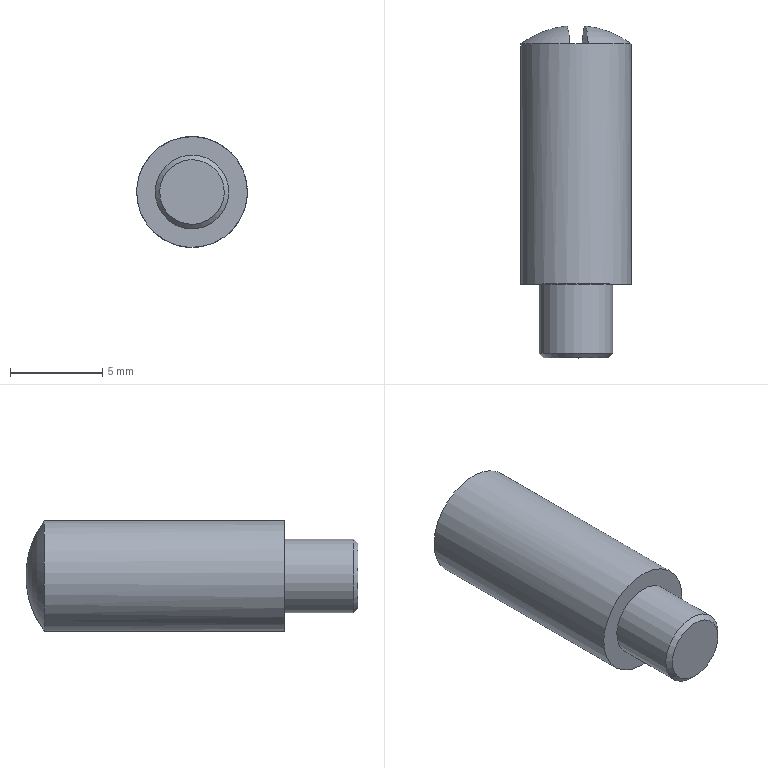Component | NX | CONN_PIN | 1 solid | 10 faces | box 6 x 17.97 x 6 mm | volume 428 mm3 | plane 5 | sphere 2 | cylinder 2 | cone 1 | commonest cylinder face diameters 4 x1 6 x1
STEP:
#1=CARTESIAN_POINT('',(0.,0.,0.));
#2=DIRECTION('',(0.,0.,1.));
#3=DIRECTION('',(1.,0.,0.));
#4=AXIS2_PLACEMENT_3D('',#1,#2,#3);
#5=CARTESIAN_POINT('',(-0.6646,-1.5,87.196));
#6=VERTEX_POINT('',#5);
#7=CARTESIAN_POINT('',(-0.3339,-1.5,93.103));
#8=VERTEX_POINT('',#7);
#9=CARTESIAN_POINT('',(-0.4992,-5.5,90.149));
#10=DIRECTION('',(0.9984,0.,-0.05589));
#11=DIRECTION('',(0.05589,0.,0.9984));
#12=AXIS2_PLACEMENT_3D('',#9,#10,#11);
#13=CIRCLE('',#12,4.975);
#14=CARTESIAN_POINT('',(-0.,-5.5,90.121));
#15=DIRECTION('',(-0.,1.,0.));
#16=DIRECTION('',(-0.05589,-0.,-0.9984));
#17=AXIS2_PLACEMENT_3D('',#14,#15,#16);
#18=SPHERICAL_SURFACE('',#17,5.);
#19=CARTESIAN_POINT('',(0.1674,0.9273));
#20=CARTESIAN_POINT('',(0.1718,0.9463));
#21=CARTESIAN_POINT('',(0.1811,0.9843));
#22=CARTESIAN_POINT('',(0.1985,1.041));
#23=CARTESIAN_POINT('',(0.2203,1.098));
#24=CARTESIAN_POINT('',(0.2482,1.154));
#25=CARTESIAN_POINT('',(0.2849,1.21));
#26=CARTESIAN_POINT('',(0.335,1.265));
#27=CARTESIAN_POINT('',(0.4066,1.319));
#28=CARTESIAN_POINT('',(0.5152,1.371));
#29=CARTESIAN_POINT('',(0.6936,1.419));
#30=CARTESIAN_POINT('',(1.007,1.459));
#31=CARTESIAN_POINT('',(1.571,1.477));
#32=CARTESIAN_POINT('',(2.135,1.459));
#33=CARTESIAN_POINT('',(2.448,1.419));
#34=CARTESIAN_POINT('',(2.626,1.371));
#35=CARTESIAN_POINT('',(2.735,1.319));
#36=CARTESIAN_POINT('',(2.807,1.265));
#37=CARTESIAN_POINT('',(2.857,1.21));
#38=CARTESIAN_POINT('',(2.893,1.154));
#39=CARTESIAN_POINT('',(2.921,1.098));
#40=CARTESIAN_POINT('',(2.943,1.041));
#41=CARTESIAN_POINT('',(2.96,0.9843));
#42=CARTESIAN_POINT('',(2.97,0.9463));
#43=CARTESIAN_POINT('',(2.974,0.9273));
#44=B_SPLINE_CURVE_WITH_KNOTS('',3,(#19,#20,#21,#22,#23,#24,#25,#26,#27,#28,#29,#30,#31,#32,#33,#34,#35,#36,#37,#38,#39,#40,#41,#42,#43),.UNSPECIFIED.,.F.,.F.,(4,1,1,1,1,1,1,1,1,1,1,1,1,1,1,1,1,1,1,1,1,1,4),(4.076,4.134,4.191,4.249,4.307,4.365,4.423,4.481,4.539,4.597,4.655,4.712,4.77,4.828,4.886,4.944,5.002,5.06,5.118,5.175,5.233,5.291,5.349),.QUASI_UNIFORM_KNOTS.);
#45=(GEOMETRIC_REPRESENTATION_CONTEXT(2)PARAMETRIC_REPRESENTATION_CONTEXT()REPRESENTATION_CONTEXT('',''));
#46=DEFINITIONAL_REPRESENTATION('',(#44),#45);
#47=PCURVE('',#18,#46);
#48=CARTESIAN_POINT('',(-0.1791,-0.5,95.868));
#49=DIRECTION('',(-0.9984,0.,0.05589));
#50=DIRECTION('',(0.05589,0.,0.9984));
#51=AXIS2_PLACEMENT_3D('',#48,#49,#50);
#52=PLANE('',#51);
#53=CARTESIAN_POINT('',(-0.7532,-5.));
#54=CARTESIAN_POINT('',(-0.7532,-13.617));
#55=CARTESIAN_POINT('',(-8.216,-9.308));
#56=CARTESIAN_POINT('',(-15.678,-5.));
#57=CARTESIAN_POINT('',(-8.216,-0.6916));
#58=CARTESIAN_POINT('',(-0.7532,3.617));
#59=CARTESIAN_POINT('',(-0.7532,-5.));
#60=(BOUNDED_CURVE()B_SPLINE_CURVE(2,(#53,#54,#55,#56,#57,#58,#59),.UNSPECIFIED.,.T.,.F.)B_SPLINE_CURVE_WITH_KNOTS((1,2,2,2,2,1),(-2.094,0.,2.094,4.189,6.283,8.378),.UNSPECIFIED.)CURVE()GEOMETRIC_REPRESENTATION_ITEM()RATIONAL_B_SPLINE_CURVE((1.,0.5,1.,0.5,1.,0.5,1.))REPRESENTATION_ITEM(''));
#61=(GEOMETRIC_REPRESENTATION_CONTEXT(2)PARAMETRIC_REPRESENTATION_CONTEXT()REPRESENTATION_CONTEXT('',''));
#62=DEFINITIONAL_REPRESENTATION('',(#60),#61);
#63=PCURVE('',#52,#62);
#64=SURFACE_CURVE('',#13,(#47,#63),.PCURVE_S1.);
#65=EDGE_CURVE('',#6,#8,#64,.T.);
#66=ORIENTED_EDGE('',*,*,#65,.F.);
#67=CARTESIAN_POINT('',(-2.995,-1.5,90.289));
#68=VERTEX_POINT('',#67);
#69=CARTESIAN_POINT('',(-0.,-1.5,90.121));
#70=DIRECTION('',(0.,1.,0.));
#71=DIRECTION('',(-0.9984,0.,0.05589));
#72=AXIS2_PLACEMENT_3D('',#69,#70,#71);
#73=CIRCLE('',#72,3.);
#74=CARTESIAN_POINT('',(-4.712,0.9273));
#75=DIRECTION('',(1.,0.));
#76=VECTOR('',#75,1.);
#77=LINE('',#74,#76);
#78=(GEOMETRIC_REPRESENTATION_CONTEXT(2)PARAMETRIC_REPRESENTATION_CONTEXT()REPRESENTATION_CONTEXT('',''));
#79=DEFINITIONAL_REPRESENTATION('',(#77),#78);
#80=PCURVE('',#18,#79);
#81=CARTESIAN_POINT('',(-0.,-14.5,90.121));
#82=DIRECTION('',(0.,1.,0.));
#83=DIRECTION('',(-0.9984,0.,0.05589));
#84=AXIS2_PLACEMENT_3D('',#81,#82,#83);
#85=CYLINDRICAL_SURFACE('',#84,3.);
#86=CARTESIAN_POINT('',(0.,13.));
#87=DIRECTION('',(1.,0.));
#88=VECTOR('',#87,1.);
#89=LINE('',#86,#88);
#90=(GEOMETRIC_REPRESENTATION_CONTEXT(2)PARAMETRIC_REPRESENTATION_CONTEXT()REPRESENTATION_CONTEXT('',''));
#91=DEFINITIONAL_REPRESENTATION('',(#89),#90);
#92=PCURVE('',#85,#91);
#93=SURFACE_CURVE('',#73,(#80,#92),.PCURVE_S1.);
#94=EDGE_CURVE('',#6,#68,#93,.T.);
#95=ORIENTED_EDGE('',*,*,#94,.T.);
#96=CARTESIAN_POINT('',(-0.,-1.5,90.121));
#97=DIRECTION('',(0.,1.,0.));
#98=DIRECTION('',(-0.9984,0.,0.05589));
#99=AXIS2_PLACEMENT_3D('',#96,#97,#98);
#100=CIRCLE('',#99,3.);
#101=CARTESIAN_POINT('',(-4.712,0.9273));
#102=DIRECTION('',(1.,0.));
#103=VECTOR('',#102,1.);
#104=LINE('',#101,#103);
#105=(GEOMETRIC_REPRESENTATION_CONTEXT(2)PARAMETRIC_REPRESENTATION_CONTEXT()REPRESENTATION_CONTEXT('',''));
#106=DEFINITIONAL_REPRESENTATION('',(#104),#105);
#107=PCURVE('',#18,#106);
#108=CARTESIAN_POINT('',(-6.283,13.));
#109=DIRECTION('',(1.,0.));
#110=VECTOR('',#109,1.);
#111=LINE('',#108,#110);
#112=(GEOMETRIC_REPRESENTATION_CONTEXT(2)PARAMETRIC_REPRESENTATION_CONTEXT()REPRESENTATION_CONTEXT('',''));
#113=DEFINITIONAL_REPRESENTATION('',(#111),#112);
#114=PCURVE('',#85,#113);
#115=SURFACE_CURVE('',#100,(#107,#114),.PCURVE_S1.);
#116=EDGE_CURVE('',#68,#8,#115,.T.);
#117=ORIENTED_EDGE('',*,*,#116,.T.);
#118=EDGE_LOOP('',(#66,#95,#117));
#119=FACE_BOUND('',#118,.T.);
#120=ADVANCED_FACE('',(#119),#18,.T.);
#121=CARTESIAN_POINT('',(1.747,-18.5,90.023));
#122=VERTEX_POINT('',#121);
#123=CARTESIAN_POINT('',(-0.,-18.5,90.121));
#124=DIRECTION('',(0.,-1.,0.));
#125=DIRECTION('',(0.9984,0.,-0.05589));
#126=AXIS2_PLACEMENT_3D('',#123,#124,#125);
#127=CIRCLE('',#126,1.75);
#128=CARTESIAN_POINT('',(-0.,-18.5,90.121));
#129=DIRECTION('',(0.,-1.,0.));
#130=DIRECTION('',(0.9984,0.,-0.05589));
#131=AXIS2_PLACEMENT_3D('',#128,#129,#130);
#132=PLANE('',#131);
#133=CARTESIAN_POINT('',(0.,0.));
#134=DIRECTION('',(1.,0.));
#135=AXIS2_PLACEMENT_2D('',#133,#134);
#136=CIRCLE('',#135,1.75);
#137=(GEOMETRIC_REPRESENTATION_CONTEXT(2)PARAMETRIC_REPRESENTATION_CONTEXT()REPRESENTATION_CONTEXT('',''));
#138=DEFINITIONAL_REPRESENTATION('',(#136),#137);
#139=PCURVE('',#132,#138);
#140=CARTESIAN_POINT('',(-0.,-18.25,90.121));
#141=DIRECTION('',(0.,1.,0.));
#142=DIRECTION('',(-0.9984,0.,0.05589));
#143=AXIS2_PLACEMENT_3D('',#140,#141,#142);
#144=CONICAL_SURFACE('',#143,2.,0.7854);
#145=CARTESIAN_POINT('',(9.425,-0.25));
#146=DIRECTION('',(-1.,0.));
#147=VECTOR('',#146,1.);
#148=LINE('',#145,#147);
#149=(GEOMETRIC_REPRESENTATION_CONTEXT(2)PARAMETRIC_REPRESENTATION_CONTEXT()REPRESENTATION_CONTEXT('',''));
#150=DEFINITIONAL_REPRESENTATION('',(#148),#149);
#151=PCURVE('',#144,#150);
#152=SURFACE_CURVE('',#127,(#139,#151),.PCURVE_S1.);
#153=EDGE_CURVE('',#122,#122,#152,.T.);
#154=ORIENTED_EDGE('',*,*,#153,.T.);
#155=EDGE_LOOP('',(#154));
#156=FACE_BOUND('',#155,.T.);
#157=ADVANCED_FACE('',(#156),#132,.T.);
#158=CARTESIAN_POINT('',(1.997,-18.25,90.009));
#159=VERTEX_POINT('',#158);
#160=CARTESIAN_POINT('',(-1.997,-18.25,90.233));
#161=VERTEX_POINT('',#160);
#162=CARTESIAN_POINT('',(-0.,-18.25,90.121));
#163=DIRECTION('',(0.,1.,0.));
#164=DIRECTION('',(0.9984,0.,-0.05589));
#165=AXIS2_PLACEMENT_3D('',#162,#163,#164);
#166=CIRCLE('',#165,2.);
#167=CARTESIAN_POINT('',(-0.,-18.5,90.121));
#168=DIRECTION('',(0.,1.,0.));
#169=DIRECTION('',(-0.9984,0.,0.05589));
#170=AXIS2_PLACEMENT_3D('',#167,#168,#169);
#171=CYLINDRICAL_SURFACE('',#170,2.);
#172=CARTESIAN_POINT('',(3.142,0.25));
#173=DIRECTION('',(1.,0.));
#174=VECTOR('',#173,1.);
#175=LINE('',#172,#174);
#176=(GEOMETRIC_REPRESENTATION_CONTEXT(2)PARAMETRIC_REPRESENTATION_CONTEXT()REPRESENTATION_CONTEXT('',''));
#177=DEFINITIONAL_REPRESENTATION('',(#175),#176);
#178=PCURVE('',#171,#177);
#179=CARTESIAN_POINT('',(3.142,-0.));
#180=DIRECTION('',(1.,0.));
#181=VECTOR('',#180,1.);
#182=LINE('',#179,#181);
#183=(GEOMETRIC_REPRESENTATION_CONTEXT(2)PARAMETRIC_REPRESENTATION_CONTEXT()REPRESENTATION_CONTEXT('',''));
#184=DEFINITIONAL_REPRESENTATION('',(#182),#183);
#185=PCURVE('',#144,#184);
#186=SURFACE_CURVE('',#166,(#178,#185),.PCURVE_S1.);
#187=EDGE_CURVE('',#159,#161,#186,.T.);
#188=ORIENTED_EDGE('',*,*,#187,.T.);
#189=CARTESIAN_POINT('',(-1.997,-14.5,90.233));
#190=VERTEX_POINT('',#189);
#191=CARTESIAN_POINT('',(-1.997,-18.25,90.233));
#192=CARTESIAN_POINT('',(-1.997,-14.5,90.233));
#193=B_SPLINE_CURVE_WITH_KNOTS('',1,(#191,#192),.UNSPECIFIED.,.F.,.F.,(2,2),(0.25,4.),.PIECEWISE_BEZIER_KNOTS.);
#194=CARTESIAN_POINT('',(6.283,0.));
#195=DIRECTION('',(0.,1.));
#196=VECTOR('',#195,1.);
#197=LINE('',#194,#196);
#198=(GEOMETRIC_REPRESENTATION_CONTEXT(2)PARAMETRIC_REPRESENTATION_CONTEXT()REPRESENTATION_CONTEXT('',''));
#199=DEFINITIONAL_REPRESENTATION('',(#197),#198);
#200=PCURVE('',#171,#199);
#201=CARTESIAN_POINT('',(0.,0.));
#202=DIRECTION('',(0.,1.));
#203=VECTOR('',#202,1.);
#204=LINE('',#201,#203);
#205=(GEOMETRIC_REPRESENTATION_CONTEXT(2)PARAMETRIC_REPRESENTATION_CONTEXT()REPRESENTATION_CONTEXT('',''));
#206=DEFINITIONAL_REPRESENTATION('',(#204),#205);
#207=PCURVE('',#171,#206);
#208=SEAM_CURVE('',#193,(#200,#207),.PCURVE_S1.);
#209=EDGE_CURVE('',#161,#190,#208,.T.);
#210=ORIENTED_EDGE('',*,*,#209,.T.);
#211=CARTESIAN_POINT('',(-0.,-14.5,90.121));
#212=DIRECTION('',(0.,-1.,0.));
#213=DIRECTION('',(-0.9984,0.,0.05589));
#214=AXIS2_PLACEMENT_3D('',#211,#212,#213);
#215=CIRCLE('',#214,2.);
#216=CARTESIAN_POINT('',(6.283,4.));
#217=DIRECTION('',(-1.,0.));
#218=VECTOR('',#217,1.);
#219=LINE('',#216,#218);
#220=(GEOMETRIC_REPRESENTATION_CONTEXT(2)PARAMETRIC_REPRESENTATION_CONTEXT()REPRESENTATION_CONTEXT('',''));
#221=DEFINITIONAL_REPRESENTATION('',(#219),#220);
#222=PCURVE('',#171,#221);
#223=CARTESIAN_POINT('',(-0.,-14.5,90.121));
#224=DIRECTION('',(0.,-1.,0.));
#225=DIRECTION('',(0.9984,0.,-0.05589));
#226=AXIS2_PLACEMENT_3D('',#223,#224,#225);
#227=PLANE('',#226);
#228=CARTESIAN_POINT('',(-0.,-0.));
#229=DIRECTION('',(-1.,0.));
#230=AXIS2_PLACEMENT_2D('',#228,#229);
#231=CIRCLE('',#230,2.);
#232=(GEOMETRIC_REPRESENTATION_CONTEXT(2)PARAMETRIC_REPRESENTATION_CONTEXT()REPRESENTATION_CONTEXT('',''));
#233=DEFINITIONAL_REPRESENTATION('',(#231),#232);
#234=PCURVE('',#227,#233);
#235=SURFACE_CURVE('',#215,(#222,#234),.PCURVE_S1.);
#236=EDGE_CURVE('',#190,#190,#235,.T.);
#237=ORIENTED_EDGE('',*,*,#236,.T.);
#238=ORIENTED_EDGE('',*,*,#209,.F.);
#239=CARTESIAN_POINT('',(-0.,-18.25,90.121));
#240=DIRECTION('',(0.,1.,0.));
#241=DIRECTION('',(0.9984,0.,-0.05589));
#242=AXIS2_PLACEMENT_3D('',#239,#240,#241);
#243=CIRCLE('',#242,2.);
#244=CARTESIAN_POINT('',(-3.142,0.25));
#245=DIRECTION('',(1.,0.));
#246=VECTOR('',#245,1.);
#247=LINE('',#244,#246);
#248=(GEOMETRIC_REPRESENTATION_CONTEXT(2)PARAMETRIC_REPRESENTATION_CONTEXT()REPRESENTATION_CONTEXT('',''));
#249=DEFINITIONAL_REPRESENTATION('',(#247),#248);
#250=PCURVE('',#171,#249);
#251=CARTESIAN_POINT('',(3.142,0.));
#252=DIRECTION('',(1.,-0.));
#253=VECTOR('',#252,1.);
#254=LINE('',#251,#253);
#255=(GEOMETRIC_REPRESENTATION_CONTEXT(2)PARAMETRIC_REPRESENTATION_CONTEXT()REPRESENTATION_CONTEXT('',''));
#256=DEFINITIONAL_REPRESENTATION('',(#254),#255);
#257=PCURVE('',#144,#256);
#258=SURFACE_CURVE('',#243,(#250,#257),.PCURVE_S1.);
#259=EDGE_CURVE('',#161,#159,#258,.T.);
#260=ORIENTED_EDGE('',*,*,#259,.T.);
#261=EDGE_LOOP('',(#188,#210,#237,#238,#260));
#262=FACE_BOUND('',#261,.T.);
#263=ADVANCED_FACE('',(#262),#171,.T.);
#264=ORIENTED_EDGE('',*,*,#236,.F.);
#265=EDGE_LOOP('',(#264));
#266=FACE_BOUND('',#265,.T.);
#267=CARTESIAN_POINT('',(-2.995,-14.5,90.289));
#268=VERTEX_POINT('',#267);
#269=CARTESIAN_POINT('',(-0.,-14.5,90.121));
#270=DIRECTION('',(0.,1.,0.));
#271=DIRECTION('',(-0.9984,0.,0.05589));
#272=AXIS2_PLACEMENT_3D('',#269,#270,#271);
#273=CIRCLE('',#272,3.);
#274=CARTESIAN_POINT('',(-3.,-0.));
#275=CARTESIAN_POINT('',(-3.,5.196));
#276=CARTESIAN_POINT('',(1.5,2.598));
#277=CARTESIAN_POINT('',(6.,0.));
#278=CARTESIAN_POINT('',(1.5,-2.598));
#279=CARTESIAN_POINT('',(-3.,-5.196));
#280=CARTESIAN_POINT('',(-3.,-0.));
#281=(BOUNDED_CURVE()B_SPLINE_CURVE(2,(#274,#275,#276,#277,#278,#279,#280),.UNSPECIFIED.,.T.,.F.)B_SPLINE_CURVE_WITH_KNOTS((1,2,2,2,2,1),(-2.094,0.,2.094,4.189,6.283,8.378),.UNSPECIFIED.)CURVE()GEOMETRIC_REPRESENTATION_ITEM()RATIONAL_B_SPLINE_CURVE((1.,0.5,1.,0.5,1.,0.5,1.))REPRESENTATION_ITEM(''));
#282=(GEOMETRIC_REPRESENTATION_CONTEXT(2)PARAMETRIC_REPRESENTATION_CONTEXT()REPRESENTATION_CONTEXT('',''));
#283=DEFINITIONAL_REPRESENTATION('',(#281),#282);
#284=PCURVE('',#227,#283);
#285=CARTESIAN_POINT('',(0.,0.));
#286=DIRECTION('',(1.,0.));
#287=VECTOR('',#286,1.);
#288=LINE('',#285,#287);
#289=(GEOMETRIC_REPRESENTATION_CONTEXT(2)PARAMETRIC_REPRESENTATION_CONTEXT()REPRESENTATION_CONTEXT('',''));
#290=DEFINITIONAL_REPRESENTATION('',(#288),#289);
#291=PCURVE('',#85,#290);
#292=SURFACE_CURVE('',#273,(#284,#291),.PCURVE_S1.);
#293=EDGE_CURVE('',#268,#268,#292,.T.);
#294=ORIENTED_EDGE('',*,*,#293,.F.);
#295=EDGE_LOOP('',(#294));
#296=FACE_BOUND('',#295,.T.);
#297=ADVANCED_FACE('',(#266,#296),#227,.T.);
#298=CARTESIAN_POINT('',(0.6646,-1.5,93.047));
#299=VERTEX_POINT('',#298);
#300=CARTESIAN_POINT('',(-0.,-1.5,90.121));
#301=DIRECTION('',(0.,1.,0.));
#302=DIRECTION('',(-0.9984,0.,0.05589));
#303=AXIS2_PLACEMENT_3D('',#300,#301,#302);
#304=CIRCLE('',#303,3.);
#305=CARTESIAN_POINT('',(0.,13.));
#306=DIRECTION('',(1.,0.));
#307=VECTOR('',#306,1.);
#308=LINE('',#305,#307);
#309=(GEOMETRIC_REPRESENTATION_CONTEXT(2)PARAMETRIC_REPRESENTATION_CONTEXT()REPRESENTATION_CONTEXT('',''));
#310=DEFINITIONAL_REPRESENTATION('',(#308),#309);
#311=PCURVE('',#85,#310);
#312=CARTESIAN_POINT('',(-0.,-1.5,90.121));
#313=DIRECTION('',(0.,-1.,0.));
#314=DIRECTION('',(0.9984,0.,-0.05589));
#315=AXIS2_PLACEMENT_3D('',#312,#313,#314);
#316=PLANE('',#315);
#317=CARTESIAN_POINT('',(-3.,-0.));
#318=CARTESIAN_POINT('',(-3.,5.196));
#319=CARTESIAN_POINT('',(1.5,2.598));
#320=CARTESIAN_POINT('',(6.,0.));
#321=CARTESIAN_POINT('',(1.5,-2.598));
#322=CARTESIAN_POINT('',(-3.,-5.196));
#323=CARTESIAN_POINT('',(-3.,-0.));
#324=(BOUNDED_CURVE()B_SPLINE_CURVE(2,(#317,#318,#319,#320,#321,#322,#323),.UNSPECIFIED.,.T.,.F.)B_SPLINE_CURVE_WITH_KNOTS((1,2,2,2,2,1),(-2.094,0.,2.094,4.189,6.283,8.378),.UNSPECIFIED.)CURVE()GEOMETRIC_REPRESENTATION_ITEM()RATIONAL_B_SPLINE_CURVE((1.,0.5,1.,0.5,1.,0.5,1.))REPRESENTATION_ITEM(''));
#325=(GEOMETRIC_REPRESENTATION_CONTEXT(2)PARAMETRIC_REPRESENTATION_CONTEXT()REPRESENTATION_CONTEXT('',''));
#326=DEFINITIONAL_REPRESENTATION('',(#324),#325);
#327=PCURVE('',#316,#326);
#328=SURFACE_CURVE('',#304,(#311,#327),.PCURVE_S1.);
#329=EDGE_CURVE('',#8,#299,#328,.T.);
#330=ORIENTED_EDGE('',*,*,#329,.F.);
#331=ORIENTED_EDGE('',*,*,#116,.F.);
#332=CARTESIAN_POINT('',(-2.995,-14.5,90.289));
#333=CARTESIAN_POINT('',(-2.995,-1.5,90.289));
#334=B_SPLINE_CURVE_WITH_KNOTS('',1,(#332,#333),.UNSPECIFIED.,.F.,.F.,(2,2),(0.,13.),.PIECEWISE_BEZIER_KNOTS.);
#335=CARTESIAN_POINT('',(0.,0.));
#336=DIRECTION('',(0.,1.));
#337=VECTOR('',#336,1.);
#338=LINE('',#335,#337);
#339=(GEOMETRIC_REPRESENTATION_CONTEXT(2)PARAMETRIC_REPRESENTATION_CONTEXT()REPRESENTATION_CONTEXT('',''));
#340=DEFINITIONAL_REPRESENTATION('',(#338),#339);
#341=PCURVE('',#85,#340);
#342=CARTESIAN_POINT('',(6.283,0.));
#343=DIRECTION('',(0.,1.));
#344=VECTOR('',#343,1.);
#345=LINE('',#342,#344);
#346=(GEOMETRIC_REPRESENTATION_CONTEXT(2)PARAMETRIC_REPRESENTATION_CONTEXT()REPRESENTATION_CONTEXT('',''));
#347=DEFINITIONAL_REPRESENTATION('',(#345),#346);
#348=PCURVE('',#85,#347);
#349=SEAM_CURVE('',#334,(#341,#348),.PCURVE_S1.);
#350=EDGE_CURVE('',#268,#68,#349,.T.);
#351=ORIENTED_EDGE('',*,*,#350,.F.);
#352=ORIENTED_EDGE('',*,*,#293,.T.);
#353=ORIENTED_EDGE('',*,*,#350,.T.);
#354=ORIENTED_EDGE('',*,*,#94,.F.);
#355=CARTESIAN_POINT('',(0.3339,-1.5,87.14));
#356=VERTEX_POINT('',#355);
#357=CARTESIAN_POINT('',(-0.,-1.5,90.121));
#358=DIRECTION('',(0.,1.,0.));
#359=DIRECTION('',(-0.9984,0.,0.05589));
#360=AXIS2_PLACEMENT_3D('',#357,#358,#359);
#361=CIRCLE('',#360,3.);
#362=CARTESIAN_POINT('',(0.,13.));
#363=DIRECTION('',(1.,0.));
#364=VECTOR('',#363,1.);
#365=LINE('',#362,#364);
#366=(GEOMETRIC_REPRESENTATION_CONTEXT(2)PARAMETRIC_REPRESENTATION_CONTEXT()REPRESENTATION_CONTEXT('',''));
#367=DEFINITIONAL_REPRESENTATION('',(#365),#366);
#368=PCURVE('',#85,#367);
#369=CARTESIAN_POINT('',(-3.,-0.));
#370=CARTESIAN_POINT('',(-3.,5.196));
#371=CARTESIAN_POINT('',(1.5,2.598));
#372=CARTESIAN_POINT('',(6.,0.));
#373=CARTESIAN_POINT('',(1.5,-2.598));
#374=CARTESIAN_POINT('',(-3.,-5.196));
#375=CARTESIAN_POINT('',(-3.,-0.));
#376=(BOUNDED_CURVE()B_SPLINE_CURVE(2,(#369,#370,#371,#372,#373,#374,#375),.UNSPECIFIED.,.T.,.F.)B_SPLINE_CURVE_WITH_KNOTS((1,2,2,2,2,1),(-2.094,0.,2.094,4.189,6.283,8.378),.UNSPECIFIED.)CURVE()GEOMETRIC_REPRESENTATION_ITEM()RATIONAL_B_SPLINE_CURVE((1.,0.5,1.,0.5,1.,0.5,1.))REPRESENTATION_ITEM(''));
#377=(GEOMETRIC_REPRESENTATION_CONTEXT(2)PARAMETRIC_REPRESENTATION_CONTEXT()REPRESENTATION_CONTEXT('',''));
#378=DEFINITIONAL_REPRESENTATION('',(#376),#377);
#379=PCURVE('',#316,#378);
#380=SURFACE_CURVE('',#361,(#368,#379),.PCURVE_S1.);
#381=EDGE_CURVE('',#356,#6,#380,.T.);
#382=ORIENTED_EDGE('',*,*,#381,.F.);
#383=CARTESIAN_POINT('',(-0.,-1.5,90.121));
#384=DIRECTION('',(0.,1.,0.));
#385=DIRECTION('',(-0.9984,0.,0.05589));
#386=AXIS2_PLACEMENT_3D('',#383,#384,#385);
#387=CIRCLE('',#386,3.);
#388=CARTESIAN_POINT('',(0.,13.));
#389=DIRECTION('',(1.,0.));
#390=VECTOR('',#389,1.);
#391=LINE('',#388,#390);
#392=(GEOMETRIC_REPRESENTATION_CONTEXT(2)PARAMETRIC_REPRESENTATION_CONTEXT()REPRESENTATION_CONTEXT('',''));
#393=DEFINITIONAL_REPRESENTATION('',(#391),#392);
#394=PCURVE('',#85,#393);
#395=CARTESIAN_POINT('',(-0.,-5.5,90.121));
#396=DIRECTION('',(-0.,1.,0.));
#397=DIRECTION('',(-0.05589,-0.,-0.9984));
#398=AXIS2_PLACEMENT_3D('',#395,#396,#397);
#399=SPHERICAL_SURFACE('',#398,5.);
#400=CARTESIAN_POINT('',(1.571,0.9273));
#401=DIRECTION('',(1.,0.));
#402=VECTOR('',#401,1.);
#403=LINE('',#400,#402);
#404=(GEOMETRIC_REPRESENTATION_CONTEXT(2)PARAMETRIC_REPRESENTATION_CONTEXT()REPRESENTATION_CONTEXT('',''));
#405=DEFINITIONAL_REPRESENTATION('',(#403),#404);
#406=PCURVE('',#399,#405);
#407=SURFACE_CURVE('',#387,(#394,#406),.PCURVE_S1.);
#408=EDGE_CURVE('',#299,#356,#407,.T.);
#409=ORIENTED_EDGE('',*,*,#408,.F.);
#410=EDGE_LOOP('',(#330,#331,#351,#352,#353,#354,#382,#409));
#411=FACE_BOUND('',#410,.T.);
#412=ADVANCED_FACE('',(#411),#85,.T.);
#413=CARTESIAN_POINT('',(0.4992,-5.5,90.093));
#414=DIRECTION('',(-0.9984,0.,0.05589));
#415=DIRECTION('',(-0.05589,0.,-0.9984));
#416=AXIS2_PLACEMENT_3D('',#413,#414,#415);
#417=CIRCLE('',#416,4.975);
#418=CARTESIAN_POINT('',(3.309,0.9273));
#419=CARTESIAN_POINT('',(3.313,0.9463));
#420=CARTESIAN_POINT('',(3.323,0.9843));
#421=CARTESIAN_POINT('',(3.34,1.041));
#422=CARTESIAN_POINT('',(3.362,1.098));
#423=CARTESIAN_POINT('',(3.39,1.154));
#424=CARTESIAN_POINT('',(3.426,1.21));
#425=CARTESIAN_POINT('',(3.477,1.265));
#426=CARTESIAN_POINT('',(3.548,1.319));
#427=CARTESIAN_POINT('',(3.657,1.371));
#428=CARTESIAN_POINT('',(3.835,1.419));
#429=CARTESIAN_POINT('',(4.148,1.459));
#430=CARTESIAN_POINT('',(4.712,1.477));
#431=CARTESIAN_POINT('',(5.277,1.459));
#432=CARTESIAN_POINT('',(5.59,1.419));
#433=CARTESIAN_POINT('',(5.768,1.371));
#434=CARTESIAN_POINT('',(5.877,1.319));
#435=CARTESIAN_POINT('',(5.948,1.265));
#436=CARTESIAN_POINT('',(5.998,1.21));
#437=CARTESIAN_POINT('',(6.035,1.154));
#438=CARTESIAN_POINT('',(6.063,1.098));
#439=CARTESIAN_POINT('',(6.085,1.041));
#440=CARTESIAN_POINT('',(6.102,0.9843));
#441=CARTESIAN_POINT('',(6.111,0.9463));
#442=CARTESIAN_POINT('',(6.116,0.9273));
#443=B_SPLINE_CURVE_WITH_KNOTS('',3,(#418,#419,#420,#421,#422,#423,#424,#425,#426,#427,#428,#429,#430,#431,#432,#433,#434,#435,#436,#437,#438,#439,#440,#441,#442),.UNSPECIFIED.,.F.,.F.,(4,1,1,1,1,1,1,1,1,1,1,1,1,1,1,1,1,1,1,1,1,1,4),(4.076,4.134,4.191,4.249,4.307,4.365,4.423,4.481,4.539,4.597,4.655,4.712,4.77,4.828,4.886,4.944,5.002,5.06,5.118,5.175,5.233,5.291,5.349),.QUASI_UNIFORM_KNOTS.);
#444=(GEOMETRIC_REPRESENTATION_CONTEXT(2)PARAMETRIC_REPRESENTATION_CONTEXT()REPRESENTATION_CONTEXT('',''));
#445=DEFINITIONAL_REPRESENTATION('',(#443),#444);
#446=PCURVE('',#399,#445);
#447=CARTESIAN_POINT('',(0.1791,-0.5,84.374));
#448=DIRECTION('',(0.9984,0.,-0.05589));
#449=DIRECTION('',(-0.05589,0.,-0.9984));
#450=AXIS2_PLACEMENT_3D('',#447,#448,#449);
#451=PLANE('',#450);
#452=CARTESIAN_POINT('',(-0.7532,-5.));
#453=CARTESIAN_POINT('',(-0.7532,-13.617));
#454=CARTESIAN_POINT('',(-8.216,-9.308));
#455=CARTESIAN_POINT('',(-15.678,-5.));
#456=CARTESIAN_POINT('',(-8.216,-0.6916));
#457=CARTESIAN_POINT('',(-0.7532,3.617));
#458=CARTESIAN_POINT('',(-0.7532,-5.));
#459=(BOUNDED_CURVE()B_SPLINE_CURVE(2,(#452,#453,#454,#455,#456,#457,#458),.UNSPECIFIED.,.T.,.F.)B_SPLINE_CURVE_WITH_KNOTS((1,2,2,2,2,1),(-2.094,0.,2.094,4.189,6.283,8.378),.UNSPECIFIED.)CURVE()GEOMETRIC_REPRESENTATION_ITEM()RATIONAL_B_SPLINE_CURVE((1.,0.5,1.,0.5,1.,0.5,1.))REPRESENTATION_ITEM(''));
#460=(GEOMETRIC_REPRESENTATION_CONTEXT(2)PARAMETRIC_REPRESENTATION_CONTEXT()REPRESENTATION_CONTEXT('',''));
#461=DEFINITIONAL_REPRESENTATION('',(#459),#460);
#462=PCURVE('',#451,#461);
#463=SURFACE_CURVE('',#417,(#446,#462),.PCURVE_S1.);
#464=EDGE_CURVE('',#299,#356,#463,.T.);
#465=ORIENTED_EDGE('',*,*,#464,.F.);
#466=ORIENTED_EDGE('',*,*,#408,.T.);
#467=EDGE_LOOP('',(#465,#466));
#468=FACE_BOUND('',#467,.T.);
#469=ADVANCED_FACE('',(#468),#399,.T.);
#470=ORIENTED_EDGE('',*,*,#65,.T.);
#471=CARTESIAN_POINT('',(-0.1791,-1.5,95.868));
#472=DIRECTION('',(0.05589,0.,0.9984));
#473=VECTOR('',#472,1.);
#474=LINE('',#471,#473);
#475=CARTESIAN_POINT('',(0.,-1.));
#476=DIRECTION('',(1.,0.));
#477=VECTOR('',#476,1.);
#478=LINE('',#475,#477);
#479=(GEOMETRIC_REPRESENTATION_CONTEXT(2)PARAMETRIC_REPRESENTATION_CONTEXT()REPRESENTATION_CONTEXT('',''));
#480=DEFINITIONAL_REPRESENTATION('',(#478),#479);
#481=PCURVE('',#52,#480);
#482=CARTESIAN_POINT('',(-0.5,5.728));
#483=DIRECTION('',(-0.,1.));
#484=VECTOR('',#483,1.);
#485=LINE('',#482,#484);
#486=(GEOMETRIC_REPRESENTATION_CONTEXT(2)PARAMETRIC_REPRESENTATION_CONTEXT()REPRESENTATION_CONTEXT('',''));
#487=DEFINITIONAL_REPRESENTATION('',(#485),#486);
#488=PCURVE('',#316,#487);
#489=SURFACE_CURVE('',#474,(#481,#488),.PCURVE_S1.);
#490=EDGE_CURVE('',#6,#8,#489,.T.);
#491=ORIENTED_EDGE('',*,*,#490,.F.);
#492=EDGE_LOOP('',(#470,#491));
#493=FACE_BOUND('',#492,.T.);
#494=ADVANCED_FACE('',(#493),#52,.F.);
#495=ORIENTED_EDGE('',*,*,#464,.T.);
#496=CARTESIAN_POINT('',(0.1791,-1.5,84.374));
#497=DIRECTION('',(-0.05589,0.,-0.9984));
#498=VECTOR('',#497,1.);
#499=LINE('',#496,#498);
#500=CARTESIAN_POINT('',(0.,-1.));
#501=DIRECTION('',(1.,0.));
#502=VECTOR('',#501,1.);
#503=LINE('',#500,#502);
#504=(GEOMETRIC_REPRESENTATION_CONTEXT(2)PARAMETRIC_REPRESENTATION_CONTEXT()REPRESENTATION_CONTEXT('',''));
#505=DEFINITIONAL_REPRESENTATION('',(#503),#504);
#506=PCURVE('',#451,#505);
#507=CARTESIAN_POINT('',(0.5,-5.728));
#508=DIRECTION('',(0.,-1.));
#509=VECTOR('',#508,1.);
#510=LINE('',#507,#509);
#511=(GEOMETRIC_REPRESENTATION_CONTEXT(2)PARAMETRIC_REPRESENTATION_CONTEXT()REPRESENTATION_CONTEXT('',''));
#512=DEFINITIONAL_REPRESENTATION('',(#510),#511);
#513=PCURVE('',#316,#512);
#514=SURFACE_CURVE('',#499,(#506,#513),.PCURVE_S1.);
#515=EDGE_CURVE('',#299,#356,#514,.T.);
#516=ORIENTED_EDGE('',*,*,#515,.F.);
#517=EDGE_LOOP('',(#495,#516));
#518=FACE_BOUND('',#517,.T.);
#519=ADVANCED_FACE('',(#518),#451,.F.);
#520=ORIENTED_EDGE('',*,*,#381,.T.);
#521=ORIENTED_EDGE('',*,*,#490,.T.);
#522=ORIENTED_EDGE('',*,*,#329,.T.);
#523=ORIENTED_EDGE('',*,*,#515,.T.);
#524=EDGE_LOOP('',(#520,#521,#522,#523));
#525=FACE_BOUND('',#524,.T.);
#526=ADVANCED_FACE('',(#525),#316,.F.);
#527=ORIENTED_EDGE('',*,*,#153,.F.);
#528=CARTESIAN_POINT('',(1.747,-18.5,90.023));
#529=CARTESIAN_POINT('',(1.997,-18.25,90.009));
#530=B_SPLINE_CURVE_WITH_KNOTS('',1,(#528,#529),.UNSPECIFIED.,.F.,.F.,(2,2),(-0.3536,-0.),.PIECEWISE_BEZIER_KNOTS.);
#531=CARTESIAN_POINT('',(9.425,0.));
#532=DIRECTION('',(0.,1.));
#533=VECTOR('',#532,1.);
#534=LINE('',#531,#533);
#535=(GEOMETRIC_REPRESENTATION_CONTEXT(2)PARAMETRIC_REPRESENTATION_CONTEXT()REPRESENTATION_CONTEXT('',''));
#536=DEFINITIONAL_REPRESENTATION('',(#534),#535);
#537=PCURVE('',#144,#536);
#538=CARTESIAN_POINT('',(3.142,0.));
#539=DIRECTION('',(0.,1.));
#540=VECTOR('',#539,1.);
#541=LINE('',#538,#540);
#542=(GEOMETRIC_REPRESENTATION_CONTEXT(2)PARAMETRIC_REPRESENTATION_CONTEXT()REPRESENTATION_CONTEXT('',''));
#543=DEFINITIONAL_REPRESENTATION('',(#541),#542);
#544=PCURVE('',#144,#543);
#545=SEAM_CURVE('',#530,(#537,#544),.PCURVE_S1.);
#546=EDGE_CURVE('',#122,#159,#545,.T.);
#547=ORIENTED_EDGE('',*,*,#546,.T.);
#548=ORIENTED_EDGE('',*,*,#259,.F.);
#549=ORIENTED_EDGE('',*,*,#187,.F.);
#550=ORIENTED_EDGE('',*,*,#546,.F.);
#551=EDGE_LOOP('',(#527,#547,#548,#549,#550));
#552=FACE_BOUND('',#551,.T.);
#553=ADVANCED_FACE('',(#552),#144,.T.);
#554=CLOSED_SHELL('',(#120,#157,#263,#297,#412,#469,#494,#519,#526,#553));
#555=MANIFOLD_SOLID_BREP('',#554);
#556=(LENGTH_UNIT()NAMED_UNIT(*)SI_UNIT(.MILLI.,.METRE.));
#557=UNCERTAINTY_MEASURE_WITH_UNIT(LENGTH_MEASURE(0.000005),#556,'','');
#558=(NAMED_UNIT(*)PLANE_ANGLE_UNIT()SI_UNIT($,.RADIAN.));
#559=(NAMED_UNIT(*)SI_UNIT($,.STERADIAN.)SOLID_ANGLE_UNIT());
#560=(GEOMETRIC_REPRESENTATION_CONTEXT(3)GLOBAL_UNCERTAINTY_ASSIGNED_CONTEXT((#557))GLOBAL_UNIT_ASSIGNED_CONTEXT((#556,#558,#559))REPRESENTATION_CONTEXT('',''));
#561=ADVANCED_BREP_SHAPE_REPRESENTATION('',(#4,#555),#560);